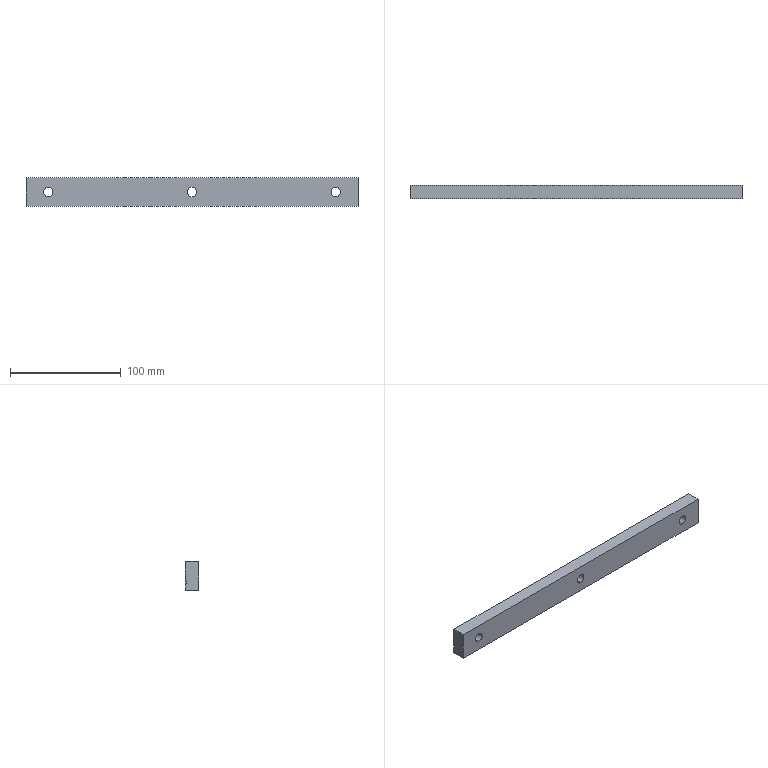Component | SolidWorks | 27RightPressurePlate-1 | 1 solid | 16 faces | box 300 x 12 x 26 mm | volume 90957 mm3 | plane 10 | cylinder 6 | commonest cylinder face diameters 8.5 x6
build123d program:
from build123d import *

# Parameters (mm, degrees)
SKETCH1_W           = 12
SKETCH1_H           = 26
BOSS_EXTRUDE1_DEPTH = 300
SKETCH2_R           = 4.25
CUT_EXTRUDE1_DEPTH  = 50
SKETCH3_W           = 2
SKETCH3_H           = 2
CUT_EXTRUDE2_DEPTH  = 5000


with BuildPart() as part:
    # Sketch1 → Boss-Extrude1 (new body)
    with BuildSketch(Plane.XY):
        Rectangle(SKETCH1_W, SKETCH1_H)
    extrude(amount=BOSS_EXTRUDE1_DEPTH)

    # Sketch2 → Cut-Extrude1 (cut)
    with BuildSketch(Plane(origin=(6, 0, 0), x_dir=(0, 0, -1), z_dir=(1, 0, 0))):
        with Locations(Location((-280, 0, 0), (0, 0, 90))):
            Circle(SKETCH2_R)
        with Locations(Location((-150, 0, 0), (0, 0, 90))):
            Circle(SKETCH2_R)
        with Locations(Location((-20, 0, 0), (0, 0, 90))):
            Circle(SKETCH2_R)
    extrude(amount=-CUT_EXTRUDE1_DEPTH, mode=Mode.SUBTRACT)

    # Sketch3 → Cut-Extrude2 (cut)
    with BuildSketch(Plane.XY.offset(300)):
        with Locations((6, -6)):
            Rectangle(SKETCH3_W, SKETCH3_H)
    extrude(amount=-CUT_EXTRUDE2_DEPTH, mode=Mode.SUBTRACT)


solid = part.part

# Placed as in the assembly
solid = solid.moved(Location((-154.717, 161, 42), (90, 90, 0)))
STEP:
#1=CARTESIAN_POINT('',(4.932,6.102,1.486));
#2=VERTEX_POINT('',#1);
#3=CARTESIAN_POINT('',(4.932,6.102,1.821));
#4=VERTEX_POINT('',#3);
#5=CARTESIAN_POINT('',(4.932,6.102,1.654));
#6=DIRECTION('',(-0.,1.,0.));
#7=DIRECTION('',(0.,0.,1.));
#8=AXIS2_PLACEMENT_3D('',#5,#6,#7);
#9=CIRCLE('',#8,0.1673);
#10=EDGE_CURVE('',#2,#4,#9,.T.);
#11=ORIENTED_EDGE('',*,*,#10,.F.);
#12=CARTESIAN_POINT('',(4.932,6.575,1.486));
#13=VERTEX_POINT('',#12);
#14=CARTESIAN_POINT('',(4.932,4.606,1.486));
#15=DIRECTION('',(-0.,1.,0.));
#16=VECTOR('',#15,39.37);
#17=LINE('',#14,#16);
#18=EDGE_CURVE('',#2,#13,#17,.T.);
#19=ORIENTED_EDGE('',*,*,#18,.T.);
#20=CARTESIAN_POINT('',(4.932,6.575,1.821));
#21=VERTEX_POINT('',#20);
#22=CARTESIAN_POINT('',(4.932,6.575,1.654));
#23=DIRECTION('',(-0.,1.,0.));
#24=DIRECTION('',(0.,0.,1.));
#25=AXIS2_PLACEMENT_3D('',#22,#23,#24);
#26=CIRCLE('',#25,0.1673);
#27=EDGE_CURVE('',#13,#21,#26,.T.);
#28=ORIENTED_EDGE('',*,*,#27,.T.);
#29=CARTESIAN_POINT('',(4.932,4.606,1.821));
#30=DIRECTION('',(-0.,1.,0.));
#31=VECTOR('',#30,39.37);
#32=LINE('',#29,#31);
#33=EDGE_CURVE('',#4,#21,#32,.T.);
#34=ORIENTED_EDGE('',*,*,#33,.F.);
#35=EDGE_LOOP('',(#11,#19,#28,#34));
#36=FACE_OUTER_BOUND('',#35,.T.);
#37=CARTESIAN_POINT('',(4.932,4.606,1.654));
#38=DIRECTION('',(-0.,1.,0.));
#39=DIRECTION('',(0.,0.,1.));
#40=AXIS2_PLACEMENT_3D('',#37,#38,#39);
#41=CYLINDRICAL_SURFACE('',#40,0.1673);
#42=ADVANCED_FACE('',(#36),#41,.F.);
#43=CARTESIAN_POINT('',(-0.1857,6.102,1.486));
#44=VERTEX_POINT('',#43);
#45=CARTESIAN_POINT('',(-0.1857,6.102,1.821));
#46=VERTEX_POINT('',#45);
#47=CARTESIAN_POINT('',(-0.1857,6.102,1.654));
#48=DIRECTION('',(-0.,1.,0.));
#49=DIRECTION('',(0.,0.,1.));
#50=AXIS2_PLACEMENT_3D('',#47,#48,#49);
#51=CIRCLE('',#50,0.1673);
#52=EDGE_CURVE('',#44,#46,#51,.T.);
#53=ORIENTED_EDGE('',*,*,#52,.F.);
#54=CARTESIAN_POINT('',(-0.1857,6.575,1.486));
#55=VERTEX_POINT('',#54);
#56=CARTESIAN_POINT('',(-0.1857,4.606,1.486));
#57=DIRECTION('',(-0.,1.,0.));
#58=VECTOR('',#57,39.37);
#59=LINE('',#56,#58);
#60=EDGE_CURVE('',#44,#55,#59,.T.);
#61=ORIENTED_EDGE('',*,*,#60,.T.);
#62=CARTESIAN_POINT('',(-0.1857,6.575,1.821));
#63=VERTEX_POINT('',#62);
#64=CARTESIAN_POINT('',(-0.1857,6.575,1.654));
#65=DIRECTION('',(-0.,1.,0.));
#66=DIRECTION('',(0.,0.,1.));
#67=AXIS2_PLACEMENT_3D('',#64,#65,#66);
#68=CIRCLE('',#67,0.1673);
#69=EDGE_CURVE('',#55,#63,#68,.T.);
#70=ORIENTED_EDGE('',*,*,#69,.T.);
#71=CARTESIAN_POINT('',(-0.1857,4.606,1.821));
#72=DIRECTION('',(-0.,1.,0.));
#73=VECTOR('',#72,39.37);
#74=LINE('',#71,#73);
#75=EDGE_CURVE('',#46,#63,#74,.T.);
#76=ORIENTED_EDGE('',*,*,#75,.F.);
#77=EDGE_LOOP('',(#53,#61,#70,#76));
#78=FACE_OUTER_BOUND('',#77,.T.);
#79=CARTESIAN_POINT('',(-0.1857,4.606,1.654));
#80=DIRECTION('',(-0.,1.,0.));
#81=DIRECTION('',(0.,0.,1.));
#82=AXIS2_PLACEMENT_3D('',#79,#80,#81);
#83=CYLINDRICAL_SURFACE('',#82,0.1673);
#84=ADVANCED_FACE('',(#78),#83,.F.);
#85=CARTESIAN_POINT('',(-5.304,6.102,1.486));
#86=VERTEX_POINT('',#85);
#87=CARTESIAN_POINT('',(-5.304,6.102,1.821));
#88=VERTEX_POINT('',#87);
#89=CARTESIAN_POINT('',(-5.304,6.102,1.654));
#90=DIRECTION('',(-0.,1.,0.));
#91=DIRECTION('',(0.,0.,1.));
#92=AXIS2_PLACEMENT_3D('',#89,#90,#91);
#93=CIRCLE('',#92,0.1673);
#94=EDGE_CURVE('',#86,#88,#93,.T.);
#95=ORIENTED_EDGE('',*,*,#94,.F.);
#96=CARTESIAN_POINT('',(-5.304,6.575,1.486));
#97=VERTEX_POINT('',#96);
#98=CARTESIAN_POINT('',(-5.304,4.606,1.486));
#99=DIRECTION('',(-0.,1.,0.));
#100=VECTOR('',#99,39.37);
#101=LINE('',#98,#100);
#102=EDGE_CURVE('',#86,#97,#101,.T.);
#103=ORIENTED_EDGE('',*,*,#102,.T.);
#104=CARTESIAN_POINT('',(-5.304,6.575,1.821));
#105=VERTEX_POINT('',#104);
#106=CARTESIAN_POINT('',(-5.304,6.575,1.654));
#107=DIRECTION('',(-0.,1.,0.));
#108=DIRECTION('',(0.,0.,1.));
#109=AXIS2_PLACEMENT_3D('',#106,#107,#108);
#110=CIRCLE('',#109,0.1673);
#111=EDGE_CURVE('',#97,#105,#110,.T.);
#112=ORIENTED_EDGE('',*,*,#111,.T.);
#113=CARTESIAN_POINT('',(-5.304,4.606,1.821));
#114=DIRECTION('',(-0.,1.,0.));
#115=VECTOR('',#114,39.37);
#116=LINE('',#113,#115);
#117=EDGE_CURVE('',#88,#105,#116,.T.);
#118=ORIENTED_EDGE('',*,*,#117,.F.);
#119=EDGE_LOOP('',(#95,#103,#112,#118));
#120=FACE_OUTER_BOUND('',#119,.T.);
#121=CARTESIAN_POINT('',(-5.304,4.606,1.654));
#122=DIRECTION('',(-0.,1.,0.));
#123=DIRECTION('',(0.,0.,1.));
#124=AXIS2_PLACEMENT_3D('',#121,#122,#123);
#125=CYLINDRICAL_SURFACE('',#124,0.1673);
#126=ADVANCED_FACE('',(#120),#125,.F.);
#127=CARTESIAN_POINT('',(-6.091,6.575,1.142));
#128=VERTEX_POINT('',#127);
#129=CARTESIAN_POINT('',(-6.091,6.575,1.378));
#130=VERTEX_POINT('',#129);
#131=CARTESIAN_POINT('',(-6.091,6.575,2.165));
#132=DIRECTION('',(0.,-0.,1.));
#133=VECTOR('',#132,39.37);
#134=LINE('',#131,#133);
#135=EDGE_CURVE('',#128,#130,#134,.T.);
#136=ORIENTED_EDGE('',*,*,#135,.T.);
#137=CARTESIAN_POINT('',(5.72,6.575,1.378));
#138=VERTEX_POINT('',#137);
#139=CARTESIAN_POINT('',(5.72,6.575,1.378));
#140=DIRECTION('',(1.,0.,-0.));
#141=VECTOR('',#140,39.37);
#142=LINE('',#139,#141);
#143=EDGE_CURVE('',#130,#138,#142,.T.);
#144=ORIENTED_EDGE('',*,*,#143,.T.);
#145=CARTESIAN_POINT('',(5.72,6.575,1.142));
#146=VERTEX_POINT('',#145);
#147=CARTESIAN_POINT('',(5.72,6.575,2.165));
#148=DIRECTION('',(0.,-0.,1.));
#149=VECTOR('',#148,39.37);
#150=LINE('',#147,#149);
#151=EDGE_CURVE('',#146,#138,#150,.T.);
#152=ORIENTED_EDGE('',*,*,#151,.F.);
#153=CARTESIAN_POINT('',(5.72,6.575,1.142));
#154=DIRECTION('',(-1.,-0.,0.));
#155=VECTOR('',#154,39.37);
#156=LINE('',#153,#155);
#157=EDGE_CURVE('',#146,#128,#156,.T.);
#158=ORIENTED_EDGE('',*,*,#157,.T.);
#159=EDGE_LOOP('',(#136,#144,#152,#158));
#160=FACE_OUTER_BOUND('',#159,.T.);
#161=CARTESIAN_POINT('',(5.72,6.575,2.165));
#162=DIRECTION('',(0.,-1.,-0.));
#163=DIRECTION('',(-0.,0.,-1.));
#164=AXIS2_PLACEMENT_3D('',#161,#162,#163);
#165=PLANE('',#164);
#166=ADVANCED_FACE('',(#160),#165,.F.);
#167=CARTESIAN_POINT('',(4.932,6.575,1.654));
#168=DIRECTION('',(-0.,1.,0.));
#169=DIRECTION('',(0.,0.,1.));
#170=AXIS2_PLACEMENT_3D('',#167,#168,#169);
#171=CIRCLE('',#170,0.1673);
#172=EDGE_CURVE('',#21,#13,#171,.T.);
#173=ORIENTED_EDGE('',*,*,#172,.F.);
#174=ORIENTED_EDGE('',*,*,#27,.F.);
#175=EDGE_LOOP('',(#173,#174));
#176=FACE_BOUND('',#175,.T.);
#177=CARTESIAN_POINT('',(-0.1857,6.575,1.654));
#178=DIRECTION('',(-0.,1.,0.));
#179=DIRECTION('',(0.,0.,1.));
#180=AXIS2_PLACEMENT_3D('',#177,#178,#179);
#181=CIRCLE('',#180,0.1673);
#182=EDGE_CURVE('',#63,#55,#181,.T.);
#183=ORIENTED_EDGE('',*,*,#182,.F.);
#184=ORIENTED_EDGE('',*,*,#69,.F.);
#185=EDGE_LOOP('',(#183,#184));
#186=FACE_BOUND('',#185,.T.);
#187=CARTESIAN_POINT('',(-5.304,6.575,1.654));
#188=DIRECTION('',(-0.,1.,0.));
#189=DIRECTION('',(0.,0.,1.));
#190=AXIS2_PLACEMENT_3D('',#187,#188,#189);
#191=CIRCLE('',#190,0.1673);
#192=EDGE_CURVE('',#105,#97,#191,.T.);
#193=ORIENTED_EDGE('',*,*,#192,.F.);
#194=ORIENTED_EDGE('',*,*,#111,.F.);
#195=EDGE_LOOP('',(#193,#194));
#196=FACE_BOUND('',#195,.T.);
#197=CARTESIAN_POINT('',(5.72,6.575,1.457));
#198=VERTEX_POINT('',#197);
#199=CARTESIAN_POINT('',(5.72,6.575,2.165));
#200=VERTEX_POINT('',#199);
#201=CARTESIAN_POINT('',(5.72,6.575,2.165));
#202=DIRECTION('',(0.,-0.,1.));
#203=VECTOR('',#202,39.37);
#204=LINE('',#201,#203);
#205=EDGE_CURVE('',#198,#200,#204,.T.);
#206=ORIENTED_EDGE('',*,*,#205,.F.);
#207=CARTESIAN_POINT('',(-6.091,6.575,1.457));
#208=VERTEX_POINT('',#207);
#209=CARTESIAN_POINT('',(5.72,6.575,1.457));
#210=DIRECTION('',(-1.,-0.,0.));
#211=VECTOR('',#210,39.37);
#212=LINE('',#209,#211);
#213=EDGE_CURVE('',#198,#208,#212,.T.);
#214=ORIENTED_EDGE('',*,*,#213,.T.);
#215=CARTESIAN_POINT('',(-6.091,6.575,2.165));
#216=VERTEX_POINT('',#215);
#217=CARTESIAN_POINT('',(-6.091,6.575,2.165));
#218=DIRECTION('',(0.,-0.,1.));
#219=VECTOR('',#218,39.37);
#220=LINE('',#217,#219);
#221=EDGE_CURVE('',#208,#216,#220,.T.);
#222=ORIENTED_EDGE('',*,*,#221,.T.);
#223=CARTESIAN_POINT('',(5.72,6.575,2.165));
#224=DIRECTION('',(-1.,-0.,0.));
#225=VECTOR('',#224,39.37);
#226=LINE('',#223,#225);
#227=EDGE_CURVE('',#200,#216,#226,.T.);
#228=ORIENTED_EDGE('',*,*,#227,.F.);
#229=EDGE_LOOP('',(#206,#214,#222,#228));
#230=FACE_OUTER_BOUND('',#229,.T.);
#231=CARTESIAN_POINT('',(5.72,6.575,2.165));
#232=DIRECTION('',(0.,-1.,-0.));
#233=DIRECTION('',(-0.,0.,-1.));
#234=AXIS2_PLACEMENT_3D('',#231,#232,#233);
#235=PLANE('',#234);
#236=ADVANCED_FACE('',(#176,#186,#196,#230),#235,.F.);
#237=CARTESIAN_POINT('',(-6.091,6.102,2.165));
#238=VERTEX_POINT('',#237);
#239=CARTESIAN_POINT('',(-6.091,6.102,2.165));
#240=DIRECTION('',(0.,-1.,-0.));
#241=VECTOR('',#240,39.37);
#242=LINE('',#239,#241);
#243=EDGE_CURVE('',#216,#238,#242,.T.);
#244=ORIENTED_EDGE('',*,*,#243,.T.);
#245=CARTESIAN_POINT('',(5.72,6.102,2.165));
#246=VERTEX_POINT('',#245);
#247=CARTESIAN_POINT('',(5.72,6.102,2.165));
#248=DIRECTION('',(-1.,-0.,0.));
#249=VECTOR('',#248,39.37);
#250=LINE('',#247,#249);
#251=EDGE_CURVE('',#246,#238,#250,.T.);
#252=ORIENTED_EDGE('',*,*,#251,.F.);
#253=CARTESIAN_POINT('',(5.72,6.102,2.165));
#254=DIRECTION('',(0.,-1.,-0.));
#255=VECTOR('',#254,39.37);
#256=LINE('',#253,#255);
#257=EDGE_CURVE('',#200,#246,#256,.T.);
#258=ORIENTED_EDGE('',*,*,#257,.F.);
#259=ORIENTED_EDGE('',*,*,#227,.T.);
#260=EDGE_LOOP('',(#244,#252,#258,#259));
#261=FACE_OUTER_BOUND('',#260,.T.);
#262=CARTESIAN_POINT('',(5.72,6.102,2.165));
#263=DIRECTION('',(-0.,0.,-1.));
#264=DIRECTION('',(-0.,1.,0.));
#265=AXIS2_PLACEMENT_3D('',#262,#263,#264);
#266=PLANE('',#265);
#267=ADVANCED_FACE('',(#261),#266,.F.);
#268=CARTESIAN_POINT('',(4.932,6.102,1.654));
#269=DIRECTION('',(-0.,1.,0.));
#270=DIRECTION('',(0.,0.,1.));
#271=AXIS2_PLACEMENT_3D('',#268,#269,#270);
#272=CIRCLE('',#271,0.1673);
#273=EDGE_CURVE('',#4,#2,#272,.T.);
#274=ORIENTED_EDGE('',*,*,#273,.T.);
#275=ORIENTED_EDGE('',*,*,#10,.T.);
#276=EDGE_LOOP('',(#274,#275));
#277=FACE_BOUND('',#276,.T.);
#278=CARTESIAN_POINT('',(-0.1857,6.102,1.654));
#279=DIRECTION('',(-0.,1.,0.));
#280=DIRECTION('',(0.,0.,1.));
#281=AXIS2_PLACEMENT_3D('',#278,#279,#280);
#282=CIRCLE('',#281,0.1673);
#283=EDGE_CURVE('',#46,#44,#282,.T.);
#284=ORIENTED_EDGE('',*,*,#283,.T.);
#285=ORIENTED_EDGE('',*,*,#52,.T.);
#286=EDGE_LOOP('',(#284,#285));
#287=FACE_BOUND('',#286,.T.);
#288=CARTESIAN_POINT('',(-5.304,6.102,1.654));
#289=DIRECTION('',(-0.,1.,0.));
#290=DIRECTION('',(0.,0.,1.));
#291=AXIS2_PLACEMENT_3D('',#288,#289,#290);
#292=CIRCLE('',#291,0.1673);
#293=EDGE_CURVE('',#88,#86,#292,.T.);
#294=ORIENTED_EDGE('',*,*,#293,.T.);
#295=ORIENTED_EDGE('',*,*,#94,.T.);
#296=EDGE_LOOP('',(#294,#295));
#297=FACE_BOUND('',#296,.T.);
#298=CARTESIAN_POINT('',(-6.091,6.102,1.142));
#299=VERTEX_POINT('',#298);
#300=CARTESIAN_POINT('',(-6.091,6.102,2.165));
#301=DIRECTION('',(-0.,0.,-1.));
#302=VECTOR('',#301,39.37);
#303=LINE('',#300,#302);
#304=EDGE_CURVE('',#238,#299,#303,.T.);
#305=ORIENTED_EDGE('',*,*,#304,.T.);
#306=CARTESIAN_POINT('',(5.72,6.102,1.142));
#307=VERTEX_POINT('',#306);
#308=CARTESIAN_POINT('',(5.72,6.102,1.142));
#309=DIRECTION('',(-1.,-0.,0.));
#310=VECTOR('',#309,39.37);
#311=LINE('',#308,#310);
#312=EDGE_CURVE('',#307,#299,#311,.T.);
#313=ORIENTED_EDGE('',*,*,#312,.F.);
#314=CARTESIAN_POINT('',(5.72,6.102,2.165));
#315=DIRECTION('',(-0.,0.,-1.));
#316=VECTOR('',#315,39.37);
#317=LINE('',#314,#316);
#318=EDGE_CURVE('',#246,#307,#317,.T.);
#319=ORIENTED_EDGE('',*,*,#318,.F.);
#320=ORIENTED_EDGE('',*,*,#251,.T.);
#321=EDGE_LOOP('',(#305,#313,#319,#320));
#322=FACE_OUTER_BOUND('',#321,.T.);
#323=CARTESIAN_POINT('',(5.72,6.102,2.165));
#324=DIRECTION('',(-0.,1.,0.));
#325=DIRECTION('',(0.,-0.,1.));
#326=AXIS2_PLACEMENT_3D('',#323,#324,#325);
#327=PLANE('',#326);
#328=ADVANCED_FACE('',(#277,#287,#297,#322),#327,.F.);
#329=CARTESIAN_POINT('',(-6.091,6.102,1.142));
#330=DIRECTION('',(-0.,1.,0.));
#331=VECTOR('',#330,39.37);
#332=LINE('',#329,#331);
#333=EDGE_CURVE('',#299,#128,#332,.T.);
#334=ORIENTED_EDGE('',*,*,#333,.T.);
#335=ORIENTED_EDGE('',*,*,#157,.F.);
#336=CARTESIAN_POINT('',(5.72,6.102,1.142));
#337=DIRECTION('',(-0.,1.,0.));
#338=VECTOR('',#337,39.37);
#339=LINE('',#336,#338);
#340=EDGE_CURVE('',#307,#146,#339,.T.);
#341=ORIENTED_EDGE('',*,*,#340,.F.);
#342=ORIENTED_EDGE('',*,*,#312,.T.);
#343=EDGE_LOOP('',(#334,#335,#341,#342));
#344=FACE_OUTER_BOUND('',#343,.T.);
#345=CARTESIAN_POINT('',(5.72,6.102,1.142));
#346=DIRECTION('',(0.,-0.,1.));
#347=DIRECTION('',(1.,0.,-0.));
#348=AXIS2_PLACEMENT_3D('',#345,#346,#347);
#349=PLANE('',#348);
#350=ADVANCED_FACE('',(#344),#349,.F.);
#351=CARTESIAN_POINT('',(5.72,6.535,1.378));
#352=VERTEX_POINT('',#351);
#353=CARTESIAN_POINT('',(5.72,6.535,1.378));
#354=DIRECTION('',(-0.,1.,0.));
#355=VECTOR('',#354,39.37);
#356=LINE('',#353,#355);
#357=EDGE_CURVE('',#352,#138,#356,.T.);
#358=ORIENTED_EDGE('',*,*,#357,.F.);
#359=CARTESIAN_POINT('',(5.72,6.535,1.457));
#360=VERTEX_POINT('',#359);
#361=CARTESIAN_POINT('',(5.72,6.535,1.457));
#362=DIRECTION('',(-0.,0.,-1.));
#363=VECTOR('',#362,39.37);
#364=LINE('',#361,#363);
#365=EDGE_CURVE('',#360,#352,#364,.T.);
#366=ORIENTED_EDGE('',*,*,#365,.F.);
#367=CARTESIAN_POINT('',(5.72,6.535,1.457));
#368=DIRECTION('',(0.,-1.,-0.));
#369=VECTOR('',#368,39.37);
#370=LINE('',#367,#369);
#371=EDGE_CURVE('',#198,#360,#370,.T.);
#372=ORIENTED_EDGE('',*,*,#371,.F.);
#373=ORIENTED_EDGE('',*,*,#205,.T.);
#374=ORIENTED_EDGE('',*,*,#257,.T.);
#375=ORIENTED_EDGE('',*,*,#318,.T.);
#376=ORIENTED_EDGE('',*,*,#340,.T.);
#377=ORIENTED_EDGE('',*,*,#151,.T.);
#378=EDGE_LOOP('',(#358,#366,#372,#373,#374,#375,#376,#377));
#379=FACE_OUTER_BOUND('',#378,.T.);
#380=CARTESIAN_POINT('',(5.72,6.339,1.654));
#381=DIRECTION('',(1.,0.,-0.));
#382=DIRECTION('',(-0.,1.,0.));
#383=AXIS2_PLACEMENT_3D('',#380,#381,#382);
#384=PLANE('',#383);
#385=ADVANCED_FACE('',(#379),#384,.T.);
#386=CARTESIAN_POINT('',(-6.091,6.535,1.457));
#387=VERTEX_POINT('',#386);
#388=CARTESIAN_POINT('',(-6.091,6.535,1.378));
#389=VERTEX_POINT('',#388);
#390=CARTESIAN_POINT('',(-6.091,6.535,1.654));
#391=DIRECTION('',(-0.,0.,-1.));
#392=VECTOR('',#391,39.37);
#393=LINE('',#390,#392);
#394=EDGE_CURVE('',#387,#389,#393,.T.);
#395=ORIENTED_EDGE('',*,*,#394,.T.);
#396=CARTESIAN_POINT('',(-6.091,6.339,1.378));
#397=DIRECTION('',(-0.,1.,0.));
#398=VECTOR('',#397,39.37);
#399=LINE('',#396,#398);
#400=EDGE_CURVE('',#389,#130,#399,.T.);
#401=ORIENTED_EDGE('',*,*,#400,.T.);
#402=ORIENTED_EDGE('',*,*,#135,.F.);
#403=ORIENTED_EDGE('',*,*,#333,.F.);
#404=ORIENTED_EDGE('',*,*,#304,.F.);
#405=ORIENTED_EDGE('',*,*,#243,.F.);
#406=ORIENTED_EDGE('',*,*,#221,.F.);
#407=CARTESIAN_POINT('',(-6.091,6.339,1.457));
#408=DIRECTION('',(0.,-1.,-0.));
#409=VECTOR('',#408,39.37);
#410=LINE('',#407,#409);
#411=EDGE_CURVE('',#208,#387,#410,.T.);
#412=ORIENTED_EDGE('',*,*,#411,.T.);
#413=EDGE_LOOP('',(#395,#401,#402,#403,#404,#405,#406,#412));
#414=FACE_OUTER_BOUND('',#413,.T.);
#415=CARTESIAN_POINT('',(-6.091,6.339,1.654));
#416=DIRECTION('',(1.,0.,-0.));
#417=DIRECTION('',(-0.,1.,0.));
#418=AXIS2_PLACEMENT_3D('',#415,#416,#417);
#419=PLANE('',#418);
#420=ADVANCED_FACE('',(#414),#419,.F.);
#421=ORIENTED_EDGE('',*,*,#102,.F.);
#422=ORIENTED_EDGE('',*,*,#293,.F.);
#423=ORIENTED_EDGE('',*,*,#117,.T.);
#424=ORIENTED_EDGE('',*,*,#192,.T.);
#425=EDGE_LOOP('',(#421,#422,#423,#424));
#426=FACE_OUTER_BOUND('',#425,.T.);
#427=CARTESIAN_POINT('',(-5.304,4.606,1.654));
#428=DIRECTION('',(-0.,1.,0.));
#429=DIRECTION('',(0.,0.,1.));
#430=AXIS2_PLACEMENT_3D('',#427,#428,#429);
#431=CYLINDRICAL_SURFACE('',#430,0.1673);
#432=ADVANCED_FACE('',(#426),#431,.F.);
#433=ORIENTED_EDGE('',*,*,#60,.F.);
#434=ORIENTED_EDGE('',*,*,#283,.F.);
#435=ORIENTED_EDGE('',*,*,#75,.T.);
#436=ORIENTED_EDGE('',*,*,#182,.T.);
#437=EDGE_LOOP('',(#433,#434,#435,#436));
#438=FACE_OUTER_BOUND('',#437,.T.);
#439=CARTESIAN_POINT('',(-0.1857,4.606,1.654));
#440=DIRECTION('',(-0.,1.,0.));
#441=DIRECTION('',(0.,0.,1.));
#442=AXIS2_PLACEMENT_3D('',#439,#440,#441);
#443=CYLINDRICAL_SURFACE('',#442,0.1673);
#444=ADVANCED_FACE('',(#438),#443,.F.);
#445=ORIENTED_EDGE('',*,*,#18,.F.);
#446=ORIENTED_EDGE('',*,*,#273,.F.);
#447=ORIENTED_EDGE('',*,*,#33,.T.);
#448=ORIENTED_EDGE('',*,*,#172,.T.);
#449=EDGE_LOOP('',(#445,#446,#447,#448));
#450=FACE_OUTER_BOUND('',#449,.T.);
#451=CARTESIAN_POINT('',(4.932,4.606,1.654));
#452=DIRECTION('',(-0.,1.,0.));
#453=DIRECTION('',(0.,0.,1.));
#454=AXIS2_PLACEMENT_3D('',#451,#452,#453);
#455=CYLINDRICAL_SURFACE('',#454,0.1673);
#456=ADVANCED_FACE('',(#450),#455,.F.);
#457=ORIENTED_EDGE('',*,*,#400,.F.);
#458=CARTESIAN_POINT('',(-191.131,6.535,1.378));
#459=DIRECTION('',(1.,0.,-0.));
#460=VECTOR('',#459,39.37);
#461=LINE('',#458,#460);
#462=EDGE_CURVE('',#389,#352,#461,.T.);
#463=ORIENTED_EDGE('',*,*,#462,.T.);
#464=ORIENTED_EDGE('',*,*,#357,.T.);
#465=ORIENTED_EDGE('',*,*,#143,.F.);
#466=EDGE_LOOP('',(#457,#463,#464,#465));
#467=FACE_OUTER_BOUND('',#466,.T.);
#468=CARTESIAN_POINT('',(-191.131,6.535,1.378));
#469=DIRECTION('',(-0.,0.,-1.));
#470=DIRECTION('',(-1.,-0.,0.));
#471=AXIS2_PLACEMENT_3D('',#468,#469,#470);
#472=PLANE('',#471);
#473=ADVANCED_FACE('',(#467),#472,.F.);
#474=CARTESIAN_POINT('',(-191.131,6.535,1.457));
#475=DIRECTION('',(1.,0.,-0.));
#476=VECTOR('',#475,39.37);
#477=LINE('',#474,#476);
#478=EDGE_CURVE('',#387,#360,#477,.T.);
#479=ORIENTED_EDGE('',*,*,#478,.T.);
#480=ORIENTED_EDGE('',*,*,#365,.T.);
#481=ORIENTED_EDGE('',*,*,#462,.F.);
#482=ORIENTED_EDGE('',*,*,#394,.F.);
#483=EDGE_LOOP('',(#479,#480,#481,#482));
#484=FACE_OUTER_BOUND('',#483,.T.);
#485=CARTESIAN_POINT('',(-191.131,6.535,1.457));
#486=DIRECTION('',(0.,-1.,-0.));
#487=DIRECTION('',(1.,0.,-0.));
#488=AXIS2_PLACEMENT_3D('',#485,#486,#487);
#489=PLANE('',#488);
#490=ADVANCED_FACE('',(#484),#489,.F.);
#491=ORIENTED_EDGE('',*,*,#371,.T.);
#492=ORIENTED_EDGE('',*,*,#478,.F.);
#493=ORIENTED_EDGE('',*,*,#411,.F.);
#494=ORIENTED_EDGE('',*,*,#213,.F.);
#495=EDGE_LOOP('',(#491,#492,#493,#494));
#496=FACE_OUTER_BOUND('',#495,.T.);
#497=CARTESIAN_POINT('',(-191.131,6.535,1.457));
#498=DIRECTION('',(0.,-0.,1.));
#499=DIRECTION('',(1.,0.,-0.));
#500=AXIS2_PLACEMENT_3D('',#497,#498,#499);
#501=PLANE('',#500);
#502=ADVANCED_FACE('',(#496),#501,.F.);
#503=CLOSED_SHELL('',(#42,#84,#126,#166,#236,#267,#328,#350,#385,#420,#432,#444,#456,#473,#490,#502));
#504=MANIFOLD_SOLID_BREP('',#503);
#505=CARTESIAN_POINT('',(0.,0.,0.));
#506=DIRECTION('',(0.,0.,1.));
#507=DIRECTION('',(1.,0.,0.));
#508=AXIS2_PLACEMENT_3D('',#505,#506,#507);
#509=(LENGTH_UNIT()NAMED_UNIT(*)SI_UNIT($,.METRE.));
#510=LENGTH_MEASURE_WITH_UNIT(LENGTH_MEASURE(0.0254),#509);
#511=DIMENSIONAL_EXPONENTS(1.,0.,0.,0.,0.,0.,0.);
#512=(CONVERSION_BASED_UNIT('',#510)LENGTH_UNIT()NAMED_UNIT(#511));
#513=UNCERTAINTY_MEASURE_WITH_UNIT(LENGTH_MEASURE(0.00001),#512,'','');
#514=(NAMED_UNIT(*)PLANE_ANGLE_UNIT()SI_UNIT($,.RADIAN.));
#515=(NAMED_UNIT(*)SI_UNIT($,.STERADIAN.)SOLID_ANGLE_UNIT());
#516=(GEOMETRIC_REPRESENTATION_CONTEXT(3)GLOBAL_UNCERTAINTY_ASSIGNED_CONTEXT((#513))GLOBAL_UNIT_ASSIGNED_CONTEXT((#512,#514,#515))REPRESENTATION_CONTEXT('',''));
#517=ADVANCED_BREP_SHAPE_REPRESENTATION('',(#504,#508),#516);
#518=COLOUR_RGB('',0.7922,0.8196,0.9333);
#519=FILL_AREA_STYLE_COLOUR('',#518);
#520=FILL_AREA_STYLE('',(#519));
#521=SURFACE_STYLE_FILL_AREA(#520);
#522=SURFACE_SIDE_STYLE('',(#521));
#523=SURFACE_STYLE_USAGE(.BOTH.,#522);
#524=PRESENTATION_STYLE_ASSIGNMENT((#523));
#525=STYLED_ITEM('',(#524),#504);
#526=(LENGTH_UNIT()NAMED_UNIT(*)SI_UNIT($,.METRE.));
#527=LENGTH_MEASURE_WITH_UNIT(LENGTH_MEASURE(0.0254),#526);
#528=DIMENSIONAL_EXPONENTS(1.,0.,0.,0.,0.,0.,0.);
#529=(CONVERSION_BASED_UNIT('',#527)LENGTH_UNIT()NAMED_UNIT(#528));
#530=UNCERTAINTY_MEASURE_WITH_UNIT(LENGTH_MEASURE(0.00001),#529,'','');
#531=(NAMED_UNIT(*)PLANE_ANGLE_UNIT()SI_UNIT($,.RADIAN.));
#532=(NAMED_UNIT(*)SI_UNIT($,.STERADIAN.)SOLID_ANGLE_UNIT());
#533=(GEOMETRIC_REPRESENTATION_CONTEXT(3)GLOBAL_UNCERTAINTY_ASSIGNED_CONTEXT((#530))GLOBAL_UNIT_ASSIGNED_CONTEXT((#529,#531,#532))REPRESENTATION_CONTEXT('',''));
#534=MECHANICAL_DESIGN_GEOMETRIC_PRESENTATION_REPRESENTATION('',(#525),#533);
#535=PRESENTATION_LAYER_ASSIGNMENT('','',(#525));